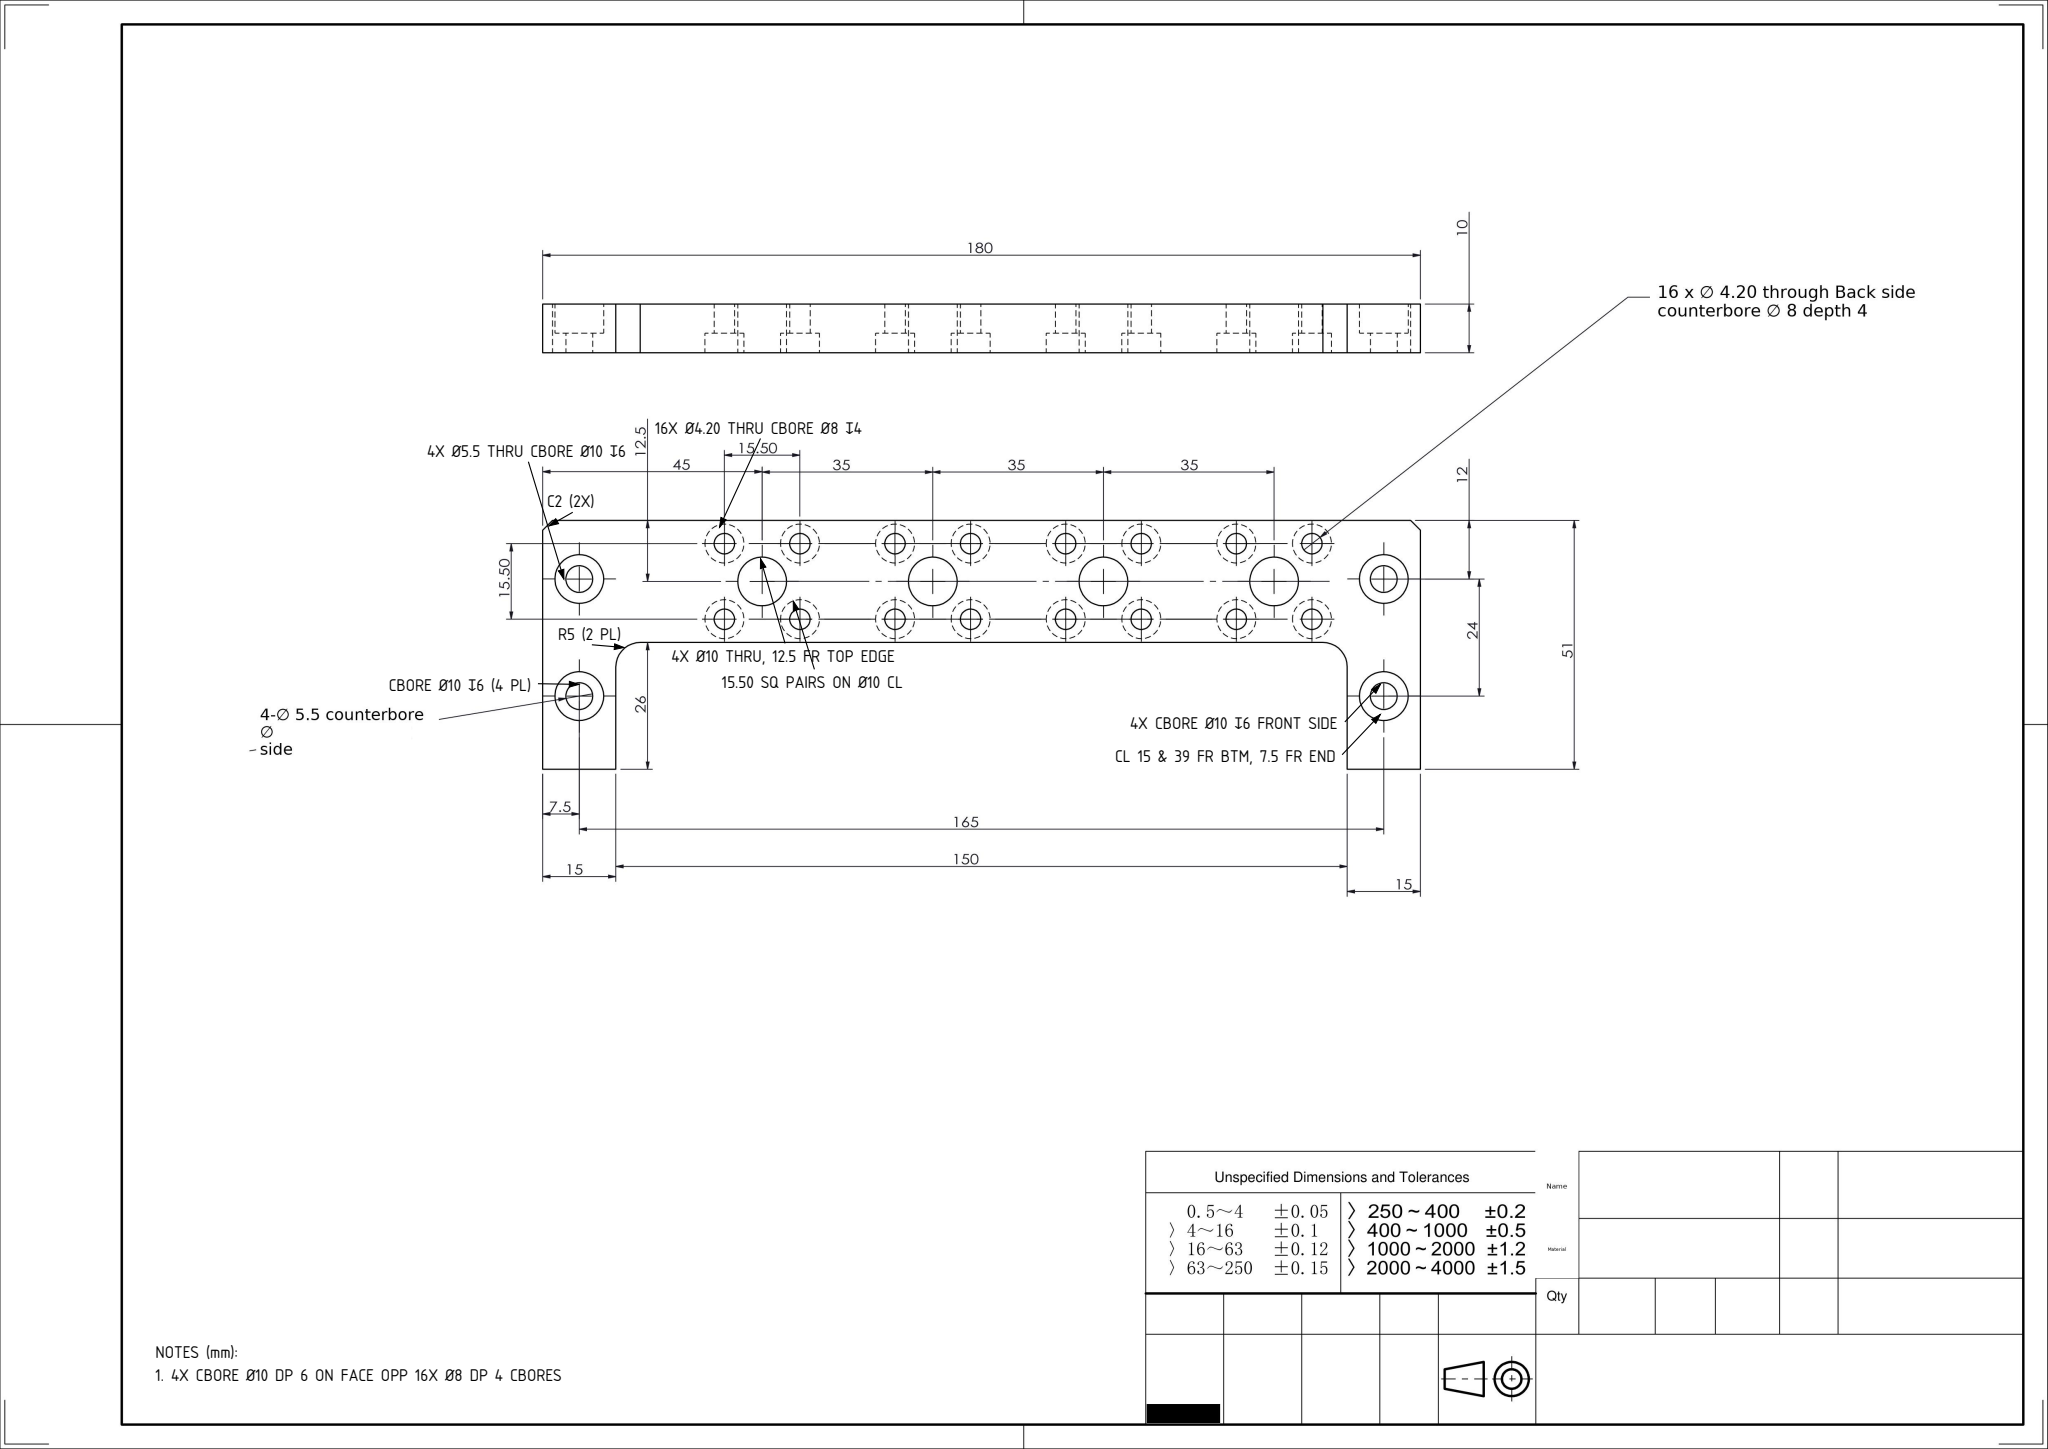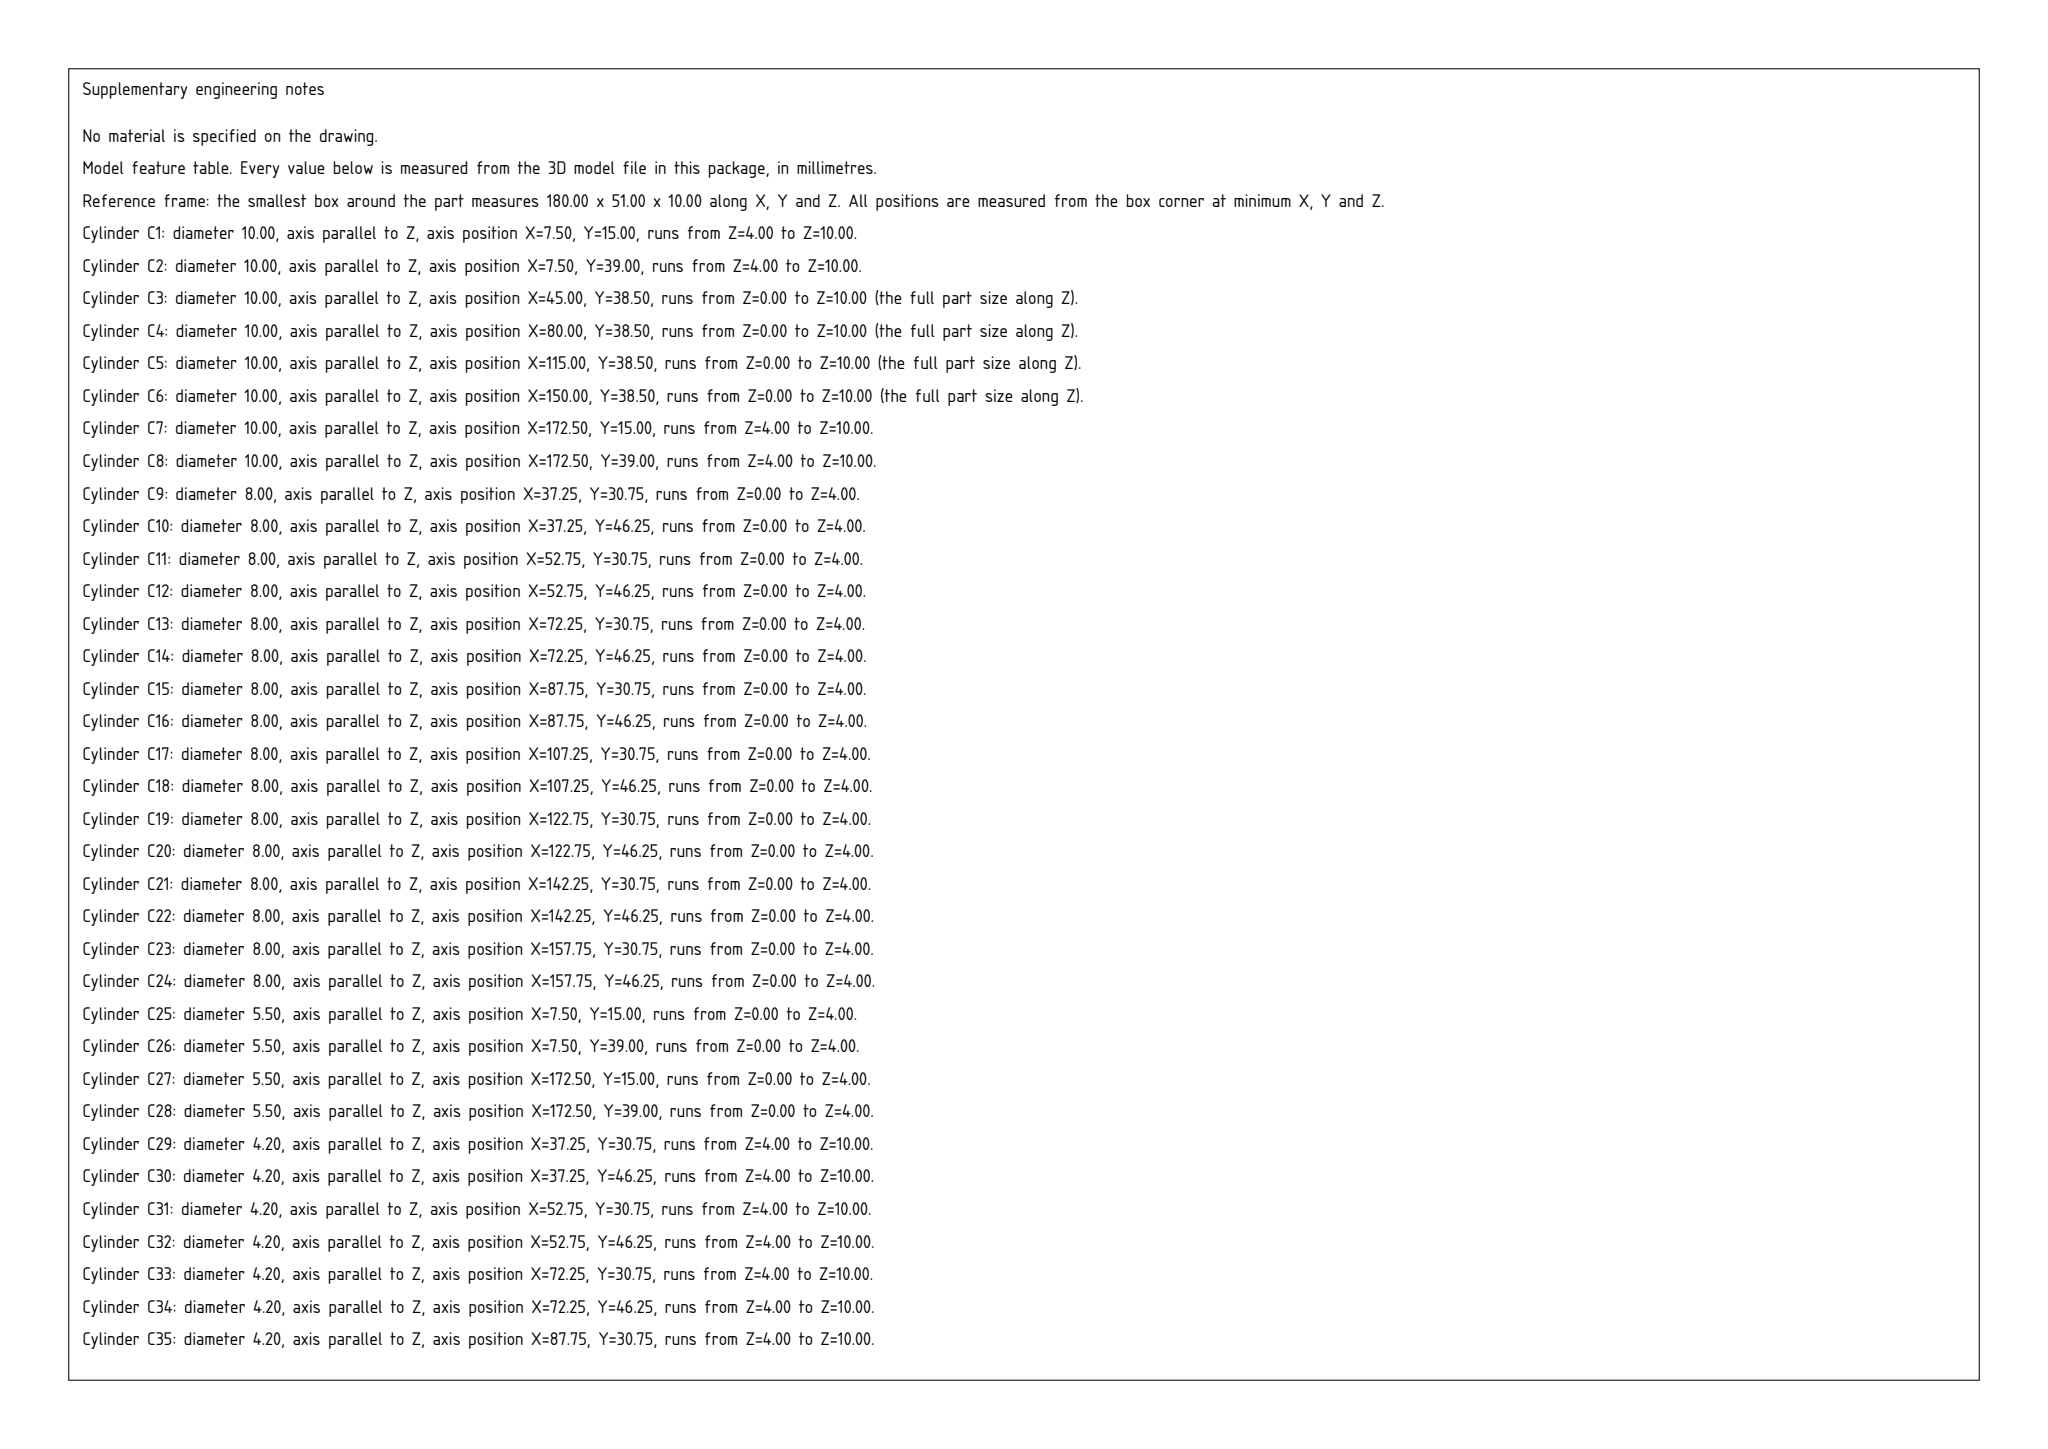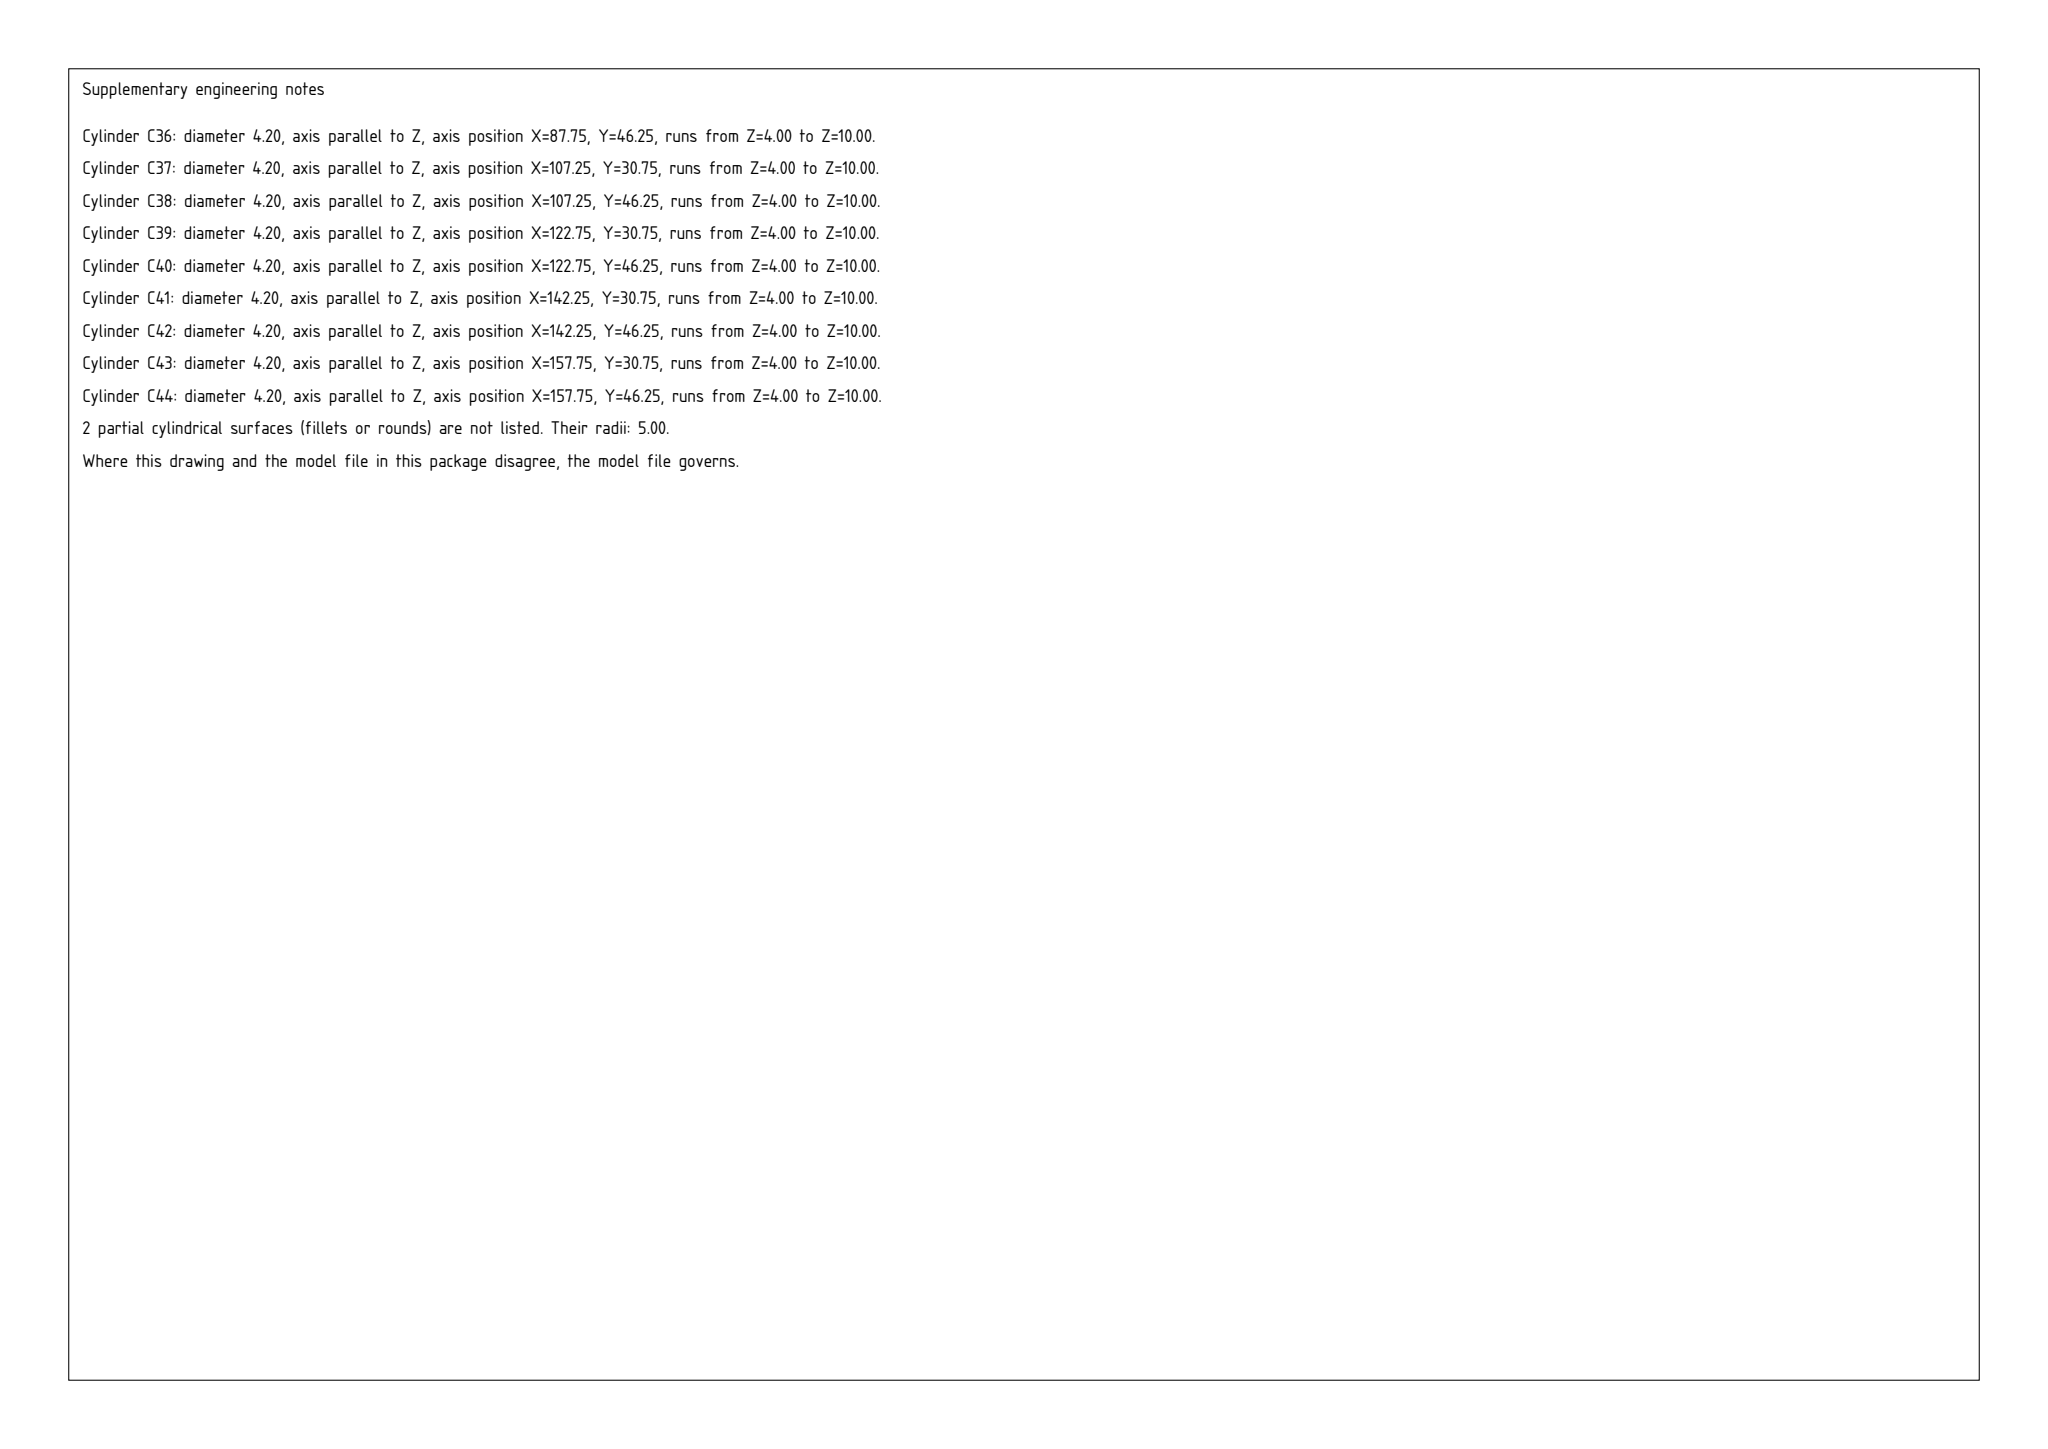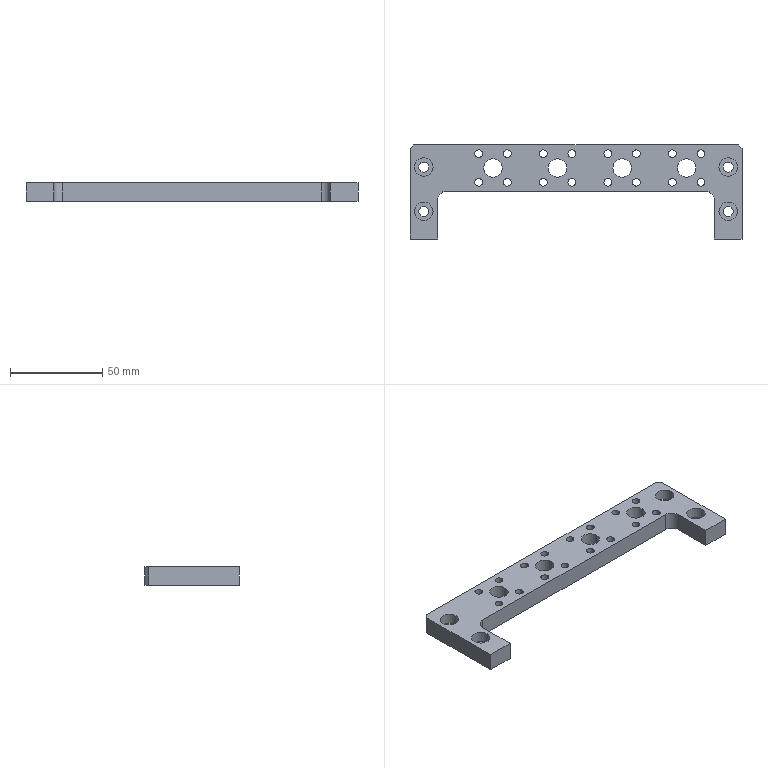Part | SolidWorks | mm | 1 solid | 122 faces | box 180 x 51 x 10 mm | volume 42914 mm3 | cylinder 90 | plane 32 | commonest cylinder face diameters 8 x32 4.2 x32 10 x18 5.5 x8
Drawing notes:
4X Ø10 THRU, CL 12.5 FR TOP EDGE, AT 45/80/115/150 | from the solid: hole/bore dia 10.0 z-axis at (45,38.5),(80,38.5),(115,38.5),(150,38.5), from 0 to 10; bbox y=51 so 51-38.5=12.5
R5 INNER FILLETS AT BOTH ENDS OF BTM NOTCH (2 PL) | from the solid: concave arcs dia 10.0 (R5), 90 deg, z-axis at (20,21) and (160,21), full 0-10 thk
C2 BOTH UPPER CORNERS (2 x 2 x 45°) | from the solid: inclined planes 45/45/90, bbox_from (0,49,0) and (178,49,0), size 2 x 2 x 10
4X Ø5.5 THRU CBORE Ø10 DP 6 FR FRONT FACE | from the solid: Ø5.5 z 0-4 and Ø10 z 4-10 at (7.5,15),(7.5,39),(172.5,15),(172.5,39); cbore 6 deep fr z=10
CBORE Ø10 DP 6, 4 PL, MEASURED FR Ø10 CBORE FACE | from the solid: Ø10 bores z 4-10 = depth 6; flat faces z=4 at 10x10 extents under the 4 corner holes
16X Ø4.20 THRU CBORE Ø8 DP 4 FR BACK FACE | from the solid: Ø4.2 z 4-10 with Ø8 z 0-4 at 16 positions; cbore flats at z=4, 8x8 extents
4X CBORE Ø10 DP 6 ON FACE OPP 16X Ø8 DP 4 CBORES | from the solid: Ø10 cbores run z 4-10 (open at z=10); Ø8 cbores run z 0-4 (open at z=0)
4X Ø5.5 THRU CBORE Ø10 DP 6, CBORE ON FRONT SIDE | from the solid: Ø5.5 z 0-4 thru to Ø10 z 4-10 at 4 corner hole positions
4X Ø5.5 CL 15 & 39 FR BTM EDGE, 7.5 FR ENDS | from the solid: Ø5.5 axes at (7.5,15),(7.5,39),(172.5,15),(172.5,39); 180-172.5=7.5
16X Ø4.20 IN 15.50 SQ PAIRS CTRD ON EA Ø10 CL | from the solid: Ø4.2 x=37.3/52.8/72.3/87.8/107.3/122.8/142.3/157.8, y=30.8/46.3; midpoints 45/80/115/150 and 38.5
build123d program:
from build123d import *

# Parameters (mm, degrees)
SKETCH1_W                                            = 180
SKETCH1_H                                            = 51
BOSS_EXTRUDE1_DEPTH                                  = 10
CUT_EXTRUDE1_DEPTH                                   = 188.353
SKETCH3_R                                            = 5
CUT_EXTRUDE2_DEPTH                                   = 188.353
HOLE_SIZE_ACCORDING_TO_THE_TYPE_OF_HEXAG_D           = 5.5
HOLE_SIZE_ACCORDING_TO_THE_TYPE_OF_HEXAG_CBORE_D     = 10
HOLE_SIZE_ACCORDING_TO_THE_TYPE_OF_HEXAG_CBORE_DEPTH = 6
F_4_2_4_2_DIAMETER_HOLE1_D                           = 4.2
SKETCH8_R                                            = 4
CUT_EXTRUDE3_DEPTH                                   = 4
LPATTERN1_COUNT                                      = 4
LPATTERN1_PITCH                                      = 35
CHAMFER1_SIZE                                        = 2


with BuildPart() as part:
    # Sketch1 → Boss-Extrude1 (new body)
    with BuildSketch(Plane.XY):
        with Locations((90, 25.5)):
            Rectangle(SKETCH1_W, SKETCH1_H)
    extrude(amount=BOSS_EXTRUDE1_DEPTH)

    # Sketch2 → Cut-Extrude1 (cut, through all)
    with BuildSketch(Plane.XY.offset(10)):
        with BuildLine():
            Line((15, 0), (165, 0))
            Line((165, 0), (165, 21))
            ThreePointArc((165, 21), (163.536, 24.536), (160, 26))
            Line((160, 26), (20, 26))
            ThreePointArc((20, 26), (16.464, 24.536), (15, 21))
            Line((15, 21), (15, 0))
        make_face()
    extrude(amount=-CUT_EXTRUDE1_DEPTH, mode=Mode.SUBTRACT)

    # Sketch3 → Cut-Extrude2 (cut, through all)
    with BuildSketch(Plane.XY.offset(10)):
        with Locations((45, 38.5)):
            Circle(SKETCH3_R)
        with Locations((80, 38.5)):
            Circle(SKETCH3_R)
        with Locations((115, 38.5)):
            Circle(SKETCH3_R)
        with Locations((150, 38.5)):
            Circle(SKETCH3_R)
    extrude(amount=-CUT_EXTRUDE2_DEPTH, mode=Mode.SUBTRACT)

    # Hole Size according to the type of Hexag (through all)
    with Locations(Plane.XY.offset(10)):
        with Locations((172.5, 39), (172.5, 15), (7.5, 15), (7.5, 39)):
            CounterBoreHole(HOLE_SIZE_ACCORDING_TO_THE_TYPE_OF_HEXAG_D / 2, HOLE_SIZE_ACCORDING_TO_THE_TYPE_OF_HEXAG_CBORE_D / 2, HOLE_SIZE_ACCORDING_TO_THE_TYPE_OF_HEXAG_CBORE_DEPTH)

    # 4.2 _4.2_ Diameter Hole1 (through all)
    with Locations(Plane.XY.offset(10)):
        with Locations((37.25, 46.25), (37.25, 30.75), (52.75, 30.75), (52.75, 46.25)):
            f_4_2_4_2_diameter_hole1 = Hole(F_4_2_4_2_DIAMETER_HOLE1_D / 2)

    # Sketch8 → Cut-Extrude3 (cut)
    with BuildSketch(Plane(origin=(0, 0, 0), x_dir=(-1, 0, 0), z_dir=(0, 0, -1))):
        with Locations((-52.75, 46.25)):
            Circle(SKETCH8_R)
        with Locations((-37.25, 46.25)):
            Circle(SKETCH8_R)
        with Locations((-37.25, 30.75)):
            Circle(SKETCH8_R)
        with Locations((-52.75, 30.75)):
            Circle(SKETCH8_R)
    cut_extrude3 = extrude(amount=-CUT_EXTRUDE3_DEPTH, mode=Mode.SUBTRACT)

    # LPattern1: 4.2 _4.2_ Diameter Hole1, Cut-Extrude3 ×4
    with Locations(*[(i * LPATTERN1_PITCH, 0, 0) for i in range(1, LPATTERN1_COUNT)]):
        add(f_4_2_4_2_diameter_hole1, mode=Mode.SUBTRACT)
        add(cut_extrude3, mode=Mode.SUBTRACT)

    # Chamfer1
    chamfer1_edges = [part.edges().sort_by_distance(p)[0] for p in [
        (0, 51, 5),
        (180, 51, 5),
    ]]
    chamfer(chamfer1_edges, length=CHAMFER1_SIZE)


solid = part.part